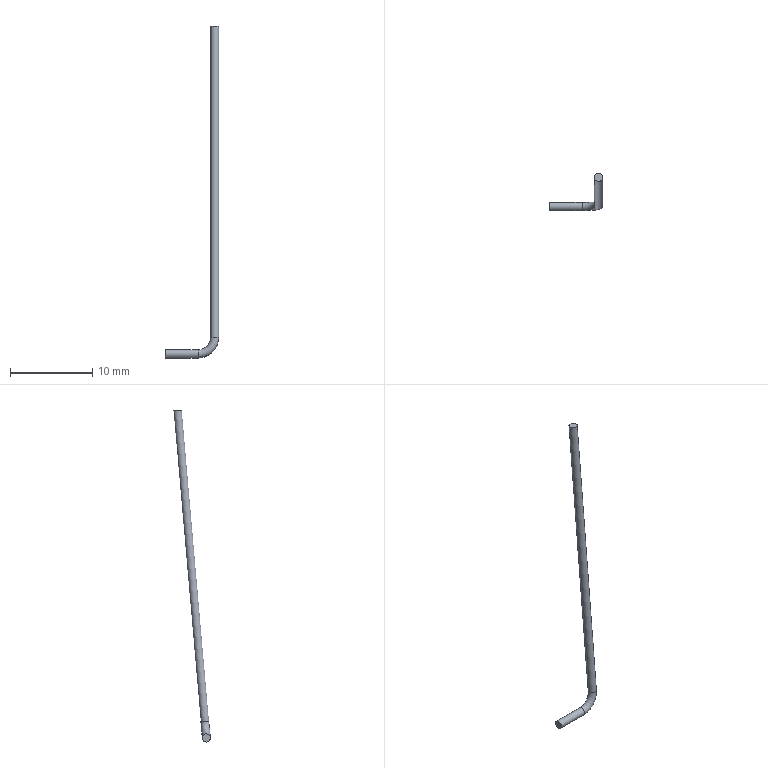Component | NX | STEPPER_WIRE | 1 solid | 5 faces | box 6.5 x 4.48 x 40.39 mm | volume 35 mm3 | cylinder 2 | plane 2 | torus 1 | commonest cylinder face diameters 1 x2
STEP:
#1=CARTESIAN_POINT('',(0.,0.,0.));
#2=DIRECTION('',(0.,0.,1.));
#3=DIRECTION('',(1.,0.,0.));
#4=AXIS2_PLACEMENT_3D('',#1,#2,#3);
#5=CARTESIAN_POINT('',(18.5,1.674,41.392));
#6=VERTEX_POINT('',#5);
#7=CARTESIAN_POINT('',(19.,1.674,41.392));
#8=DIRECTION('',(0.,0.08716,0.9962));
#9=DIRECTION('',(-1.,0.,0.));
#10=AXIS2_PLACEMENT_3D('',#7,#8,#9);
#11=CIRCLE('',#10,0.5);
#12=CARTESIAN_POINT('',(19.,1.674,41.392));
#13=DIRECTION('',(0.,0.08716,0.9962));
#14=DIRECTION('',(-1.,0.,0.));
#15=AXIS2_PLACEMENT_3D('',#12,#13,#14);
#16=CYLINDRICAL_SURFACE('',#15,0.5);
#17=CARTESIAN_POINT('',(0.,0.));
#18=DIRECTION('',(1.,0.));
#19=VECTOR('',#18,1.);
#20=LINE('',#17,#19);
#21=(GEOMETRIC_REPRESENTATION_CONTEXT(2)PARAMETRIC_REPRESENTATION_CONTEXT()REPRESENTATION_CONTEXT('',''));
#22=DEFINITIONAL_REPRESENTATION('',(#20),#21);
#23=PCURVE('',#16,#22);
#24=CARTESIAN_POINT('',(17.,1.674,41.392));
#25=DIRECTION('',(0.,-0.9962,0.08716));
#26=DIRECTION('',(1.,0.,0.));
#27=AXIS2_PLACEMENT_3D('',#24,#25,#26);
#28=TOROIDAL_SURFACE('',#27,2.,0.5);
#29=CARTESIAN_POINT('',(6.283,9.425));
#30=DIRECTION('',(0.,-1.));
#31=VECTOR('',#30,1.);
#32=LINE('',#29,#31);
#33=(GEOMETRIC_REPRESENTATION_CONTEXT(2)PARAMETRIC_REPRESENTATION_CONTEXT()REPRESENTATION_CONTEXT('',''));
#34=DEFINITIONAL_REPRESENTATION('',(#32),#33);
#35=PCURVE('',#28,#34);
#36=SURFACE_CURVE('',#11,(#23,#35),.PCURVE_S1.);
#37=EDGE_CURVE('',#6,#6,#36,.T.);
#38=ORIENTED_EDGE('',*,*,#37,.T.);
#39=CARTESIAN_POINT('',(18.5,4.986,79.248));
#40=VERTEX_POINT('',#39);
#41=CARTESIAN_POINT('',(18.5,1.674,41.392));
#42=CARTESIAN_POINT('',(18.5,4.986,79.248));
#43=B_SPLINE_CURVE_WITH_KNOTS('',1,(#41,#42),.UNSPECIFIED.,.F.,.F.,(2,2),(0.,38.),.PIECEWISE_BEZIER_KNOTS.);
#44=CARTESIAN_POINT('',(6.283,0.));
#45=DIRECTION('',(0.,1.));
#46=VECTOR('',#45,1.);
#47=LINE('',#44,#46);
#48=(GEOMETRIC_REPRESENTATION_CONTEXT(2)PARAMETRIC_REPRESENTATION_CONTEXT()REPRESENTATION_CONTEXT('',''));
#49=DEFINITIONAL_REPRESENTATION('',(#47),#48);
#50=PCURVE('',#16,#49);
#51=CARTESIAN_POINT('',(0.,0.));
#52=DIRECTION('',(0.,1.));
#53=VECTOR('',#52,1.);
#54=LINE('',#51,#53);
#55=(GEOMETRIC_REPRESENTATION_CONTEXT(2)PARAMETRIC_REPRESENTATION_CONTEXT()REPRESENTATION_CONTEXT('',''));
#56=DEFINITIONAL_REPRESENTATION('',(#54),#55);
#57=PCURVE('',#16,#56);
#58=SEAM_CURVE('',#43,(#50,#57),.PCURVE_S1.);
#59=EDGE_CURVE('',#6,#40,#58,.T.);
#60=ORIENTED_EDGE('',*,*,#59,.T.);
#61=CARTESIAN_POINT('',(19.,4.986,79.248));
#62=DIRECTION('',(0.,0.08716,0.9962));
#63=DIRECTION('',(-1.,0.,0.));
#64=AXIS2_PLACEMENT_3D('',#61,#62,#63);
#65=CIRCLE('',#64,0.5);
#66=CARTESIAN_POINT('',(0.,38.));
#67=DIRECTION('',(1.,0.));
#68=VECTOR('',#67,1.);
#69=LINE('',#66,#68);
#70=(GEOMETRIC_REPRESENTATION_CONTEXT(2)PARAMETRIC_REPRESENTATION_CONTEXT()REPRESENTATION_CONTEXT('',''));
#71=DEFINITIONAL_REPRESENTATION('',(#69),#70);
#72=PCURVE('',#16,#71);
#73=CARTESIAN_POINT('',(19.,4.986,79.248));
#74=DIRECTION('',(0.,0.08716,0.9962));
#75=DIRECTION('',(-1.,0.,0.));
#76=AXIS2_PLACEMENT_3D('',#73,#74,#75);
#77=PLANE('',#76);
#78=CARTESIAN_POINT('',(0.,0.));
#79=DIRECTION('',(1.,-0.));
#80=AXIS2_PLACEMENT_2D('',#78,#79);
#81=CIRCLE('',#80,0.5);
#82=(GEOMETRIC_REPRESENTATION_CONTEXT(2)PARAMETRIC_REPRESENTATION_CONTEXT()REPRESENTATION_CONTEXT('',''));
#83=DEFINITIONAL_REPRESENTATION('',(#81),#82);
#84=PCURVE('',#77,#83);
#85=SURFACE_CURVE('',#65,(#72,#84),.PCURVE_S1.);
#86=EDGE_CURVE('',#40,#40,#85,.T.);
#87=ORIENTED_EDGE('',*,*,#86,.F.);
#88=ORIENTED_EDGE('',*,*,#59,.F.);
#89=EDGE_LOOP('',(#38,#60,#87,#88));
#90=FACE_BOUND('',#89,.T.);
#91=ADVANCED_FACE('',(#90),#16,.T.);
#92=CARTESIAN_POINT('',(17.,1.544,39.898));
#93=VERTEX_POINT('',#92);
#94=CARTESIAN_POINT('',(17.,1.5,39.4));
#95=DIRECTION('',(1.,0.,0.));
#96=DIRECTION('',(0.,0.08716,0.9962));
#97=AXIS2_PLACEMENT_3D('',#94,#95,#96);
#98=CIRCLE('',#97,0.5);
#99=CARTESIAN_POINT('',(4.712,9.425));
#100=DIRECTION('',(0.,-1.));
#101=VECTOR('',#100,1.);
#102=LINE('',#99,#101);
#103=(GEOMETRIC_REPRESENTATION_CONTEXT(2)PARAMETRIC_REPRESENTATION_CONTEXT()REPRESENTATION_CONTEXT('',''));
#104=DEFINITIONAL_REPRESENTATION('',(#102),#103);
#105=PCURVE('',#28,#104);
#106=CARTESIAN_POINT('',(17.,1.5,39.4));
#107=DIRECTION('',(-1.,0.,0.));
#108=DIRECTION('',(0.,-0.08716,-0.9962));
#109=AXIS2_PLACEMENT_3D('',#106,#107,#108);
#110=CYLINDRICAL_SURFACE('',#109,0.5);
#111=CARTESIAN_POINT('',(9.425,0.));
#112=DIRECTION('',(-1.,0.));
#113=VECTOR('',#112,1.);
#114=LINE('',#111,#113);
#115=(GEOMETRIC_REPRESENTATION_CONTEXT(2)PARAMETRIC_REPRESENTATION_CONTEXT()REPRESENTATION_CONTEXT('',''));
#116=DEFINITIONAL_REPRESENTATION('',(#114),#115);
#117=PCURVE('',#110,#116);
#118=SURFACE_CURVE('',#98,(#105,#117),.PCURVE_S1.);
#119=EDGE_CURVE('',#93,#93,#118,.T.);
#120=ORIENTED_EDGE('',*,*,#119,.T.);
#121=CARTESIAN_POINT('',(17.,1.544,39.898));
#122=CARTESIAN_POINT('',(17.401,1.544,39.898));
#123=CARTESIAN_POINT('',(17.792,1.555,40.025));
#124=CARTESIAN_POINT('',(18.128,1.576,40.269));
#125=CARTESIAN_POINT('',(18.372,1.605,40.604));
#126=CARTESIAN_POINT('',(18.5,1.639,40.993));
#127=CARTESIAN_POINT('',(18.5,1.674,41.392));
#128=(BOUNDED_CURVE()B_SPLINE_CURVE(6,(#121,#122,#123,#124,#125,#126,#127),.UNSPECIFIED.,.F.,.F.)B_SPLINE_CURVE_WITH_KNOTS((7,7),(4.712,6.283),.PIECEWISE_BEZIER_KNOTS.)CURVE()GEOMETRIC_REPRESENTATION_ITEM()RATIONAL_B_SPLINE_CURVE((1.031,1.01,0.9979,0.994,0.9979,1.01,1.031))REPRESENTATION_ITEM(''));
#129=CARTESIAN_POINT('',(0.,3.142));
#130=DIRECTION('',(1.,0.));
#131=VECTOR('',#130,1.);
#132=LINE('',#129,#131);
#133=(GEOMETRIC_REPRESENTATION_CONTEXT(2)PARAMETRIC_REPRESENTATION_CONTEXT()REPRESENTATION_CONTEXT('',''));
#134=DEFINITIONAL_REPRESENTATION('',(#132),#133);
#135=PCURVE('',#28,#134);
#136=CARTESIAN_POINT('',(0.,9.425));
#137=DIRECTION('',(1.,0.));
#138=VECTOR('',#137,1.);
#139=LINE('',#136,#138);
#140=(GEOMETRIC_REPRESENTATION_CONTEXT(2)PARAMETRIC_REPRESENTATION_CONTEXT()REPRESENTATION_CONTEXT('',''));
#141=DEFINITIONAL_REPRESENTATION('',(#139),#140);
#142=PCURVE('',#28,#141);
#143=SEAM_CURVE('',#128,(#135,#142),.PCURVE_S1.);
#144=EDGE_CURVE('',#93,#6,#143,.T.);
#145=ORIENTED_EDGE('',*,*,#144,.T.);
#146=ORIENTED_EDGE('',*,*,#37,.F.);
#147=ORIENTED_EDGE('',*,*,#144,.F.);
#148=EDGE_LOOP('',(#120,#145,#146,#147));
#149=FACE_BOUND('',#148,.T.);
#150=ADVANCED_FACE('',(#149),#28,.T.);
#151=ORIENTED_EDGE('',*,*,#119,.F.);
#152=CARTESIAN_POINT('',(13.,1.544,39.898));
#153=VERTEX_POINT('',#152);
#154=CARTESIAN_POINT('',(17.,1.544,39.898));
#155=CARTESIAN_POINT('',(13.,1.544,39.898));
#156=B_SPLINE_CURVE_WITH_KNOTS('',1,(#154,#155),.UNSPECIFIED.,.F.,.F.,(2,2),(0.,4.),.PIECEWISE_BEZIER_KNOTS.);
#157=CARTESIAN_POINT('',(9.425,0.));
#158=DIRECTION('',(0.,1.));
#159=VECTOR('',#158,1.);
#160=LINE('',#157,#159);
#161=(GEOMETRIC_REPRESENTATION_CONTEXT(2)PARAMETRIC_REPRESENTATION_CONTEXT()REPRESENTATION_CONTEXT('',''));
#162=DEFINITIONAL_REPRESENTATION('',(#160),#161);
#163=PCURVE('',#110,#162);
#164=CARTESIAN_POINT('',(3.142,0.));
#165=DIRECTION('',(0.,1.));
#166=VECTOR('',#165,1.);
#167=LINE('',#164,#166);
#168=(GEOMETRIC_REPRESENTATION_CONTEXT(2)PARAMETRIC_REPRESENTATION_CONTEXT()REPRESENTATION_CONTEXT('',''));
#169=DEFINITIONAL_REPRESENTATION('',(#167),#168);
#170=PCURVE('',#110,#169);
#171=SEAM_CURVE('',#156,(#163,#170),.PCURVE_S1.);
#172=EDGE_CURVE('',#93,#153,#171,.T.);
#173=ORIENTED_EDGE('',*,*,#172,.T.);
#174=CARTESIAN_POINT('',(13.,1.5,39.4));
#175=DIRECTION('',(1.,0.,0.));
#176=DIRECTION('',(0.,0.08716,0.9962));
#177=AXIS2_PLACEMENT_3D('',#174,#175,#176);
#178=CIRCLE('',#177,0.5);
#179=CARTESIAN_POINT('',(9.425,4.));
#180=DIRECTION('',(-1.,0.));
#181=VECTOR('',#180,1.);
#182=LINE('',#179,#181);
#183=(GEOMETRIC_REPRESENTATION_CONTEXT(2)PARAMETRIC_REPRESENTATION_CONTEXT()REPRESENTATION_CONTEXT('',''));
#184=DEFINITIONAL_REPRESENTATION('',(#182),#183);
#185=PCURVE('',#110,#184);
#186=CARTESIAN_POINT('',(13.,1.5,39.4));
#187=DIRECTION('',(1.,0.,0.));
#188=DIRECTION('',(0.,0.08716,0.9962));
#189=AXIS2_PLACEMENT_3D('',#186,#187,#188);
#190=PLANE('',#189);
#191=CARTESIAN_POINT('',(0.,0.));
#192=DIRECTION('',(1.,-0.));
#193=AXIS2_PLACEMENT_2D('',#191,#192);
#194=CIRCLE('',#193,0.5);
#195=(GEOMETRIC_REPRESENTATION_CONTEXT(2)PARAMETRIC_REPRESENTATION_CONTEXT()REPRESENTATION_CONTEXT('',''));
#196=DEFINITIONAL_REPRESENTATION('',(#194),#195);
#197=PCURVE('',#190,#196);
#198=SURFACE_CURVE('',#178,(#185,#197),.PCURVE_S1.);
#199=EDGE_CURVE('',#153,#153,#198,.T.);
#200=ORIENTED_EDGE('',*,*,#199,.T.);
#201=ORIENTED_EDGE('',*,*,#172,.F.);
#202=EDGE_LOOP('',(#151,#173,#200,#201));
#203=FACE_BOUND('',#202,.T.);
#204=ADVANCED_FACE('',(#203),#110,.T.);
#205=ORIENTED_EDGE('',*,*,#86,.T.);
#206=EDGE_LOOP('',(#205));
#207=FACE_BOUND('',#206,.T.);
#208=ADVANCED_FACE('',(#207),#77,.T.);
#209=ORIENTED_EDGE('',*,*,#199,.F.);
#210=EDGE_LOOP('',(#209));
#211=FACE_BOUND('',#210,.T.);
#212=ADVANCED_FACE('',(#211),#190,.F.);
#213=CLOSED_SHELL('',(#91,#150,#204,#208,#212));
#214=MANIFOLD_SOLID_BREP('',#213);
#215=(LENGTH_UNIT()NAMED_UNIT(*)SI_UNIT(.MILLI.,.METRE.));
#216=UNCERTAINTY_MEASURE_WITH_UNIT(LENGTH_MEASURE(0.00001),#215,'','');
#217=(NAMED_UNIT(*)PLANE_ANGLE_UNIT()SI_UNIT($,.RADIAN.));
#218=(NAMED_UNIT(*)SI_UNIT($,.STERADIAN.)SOLID_ANGLE_UNIT());
#219=(GEOMETRIC_REPRESENTATION_CONTEXT(3)GLOBAL_UNCERTAINTY_ASSIGNED_CONTEXT((#216))GLOBAL_UNIT_ASSIGNED_CONTEXT((#215,#217,#218))REPRESENTATION_CONTEXT('',''));
#220=ADVANCED_BREP_SHAPE_REPRESENTATION('',(#4,#214),#219);